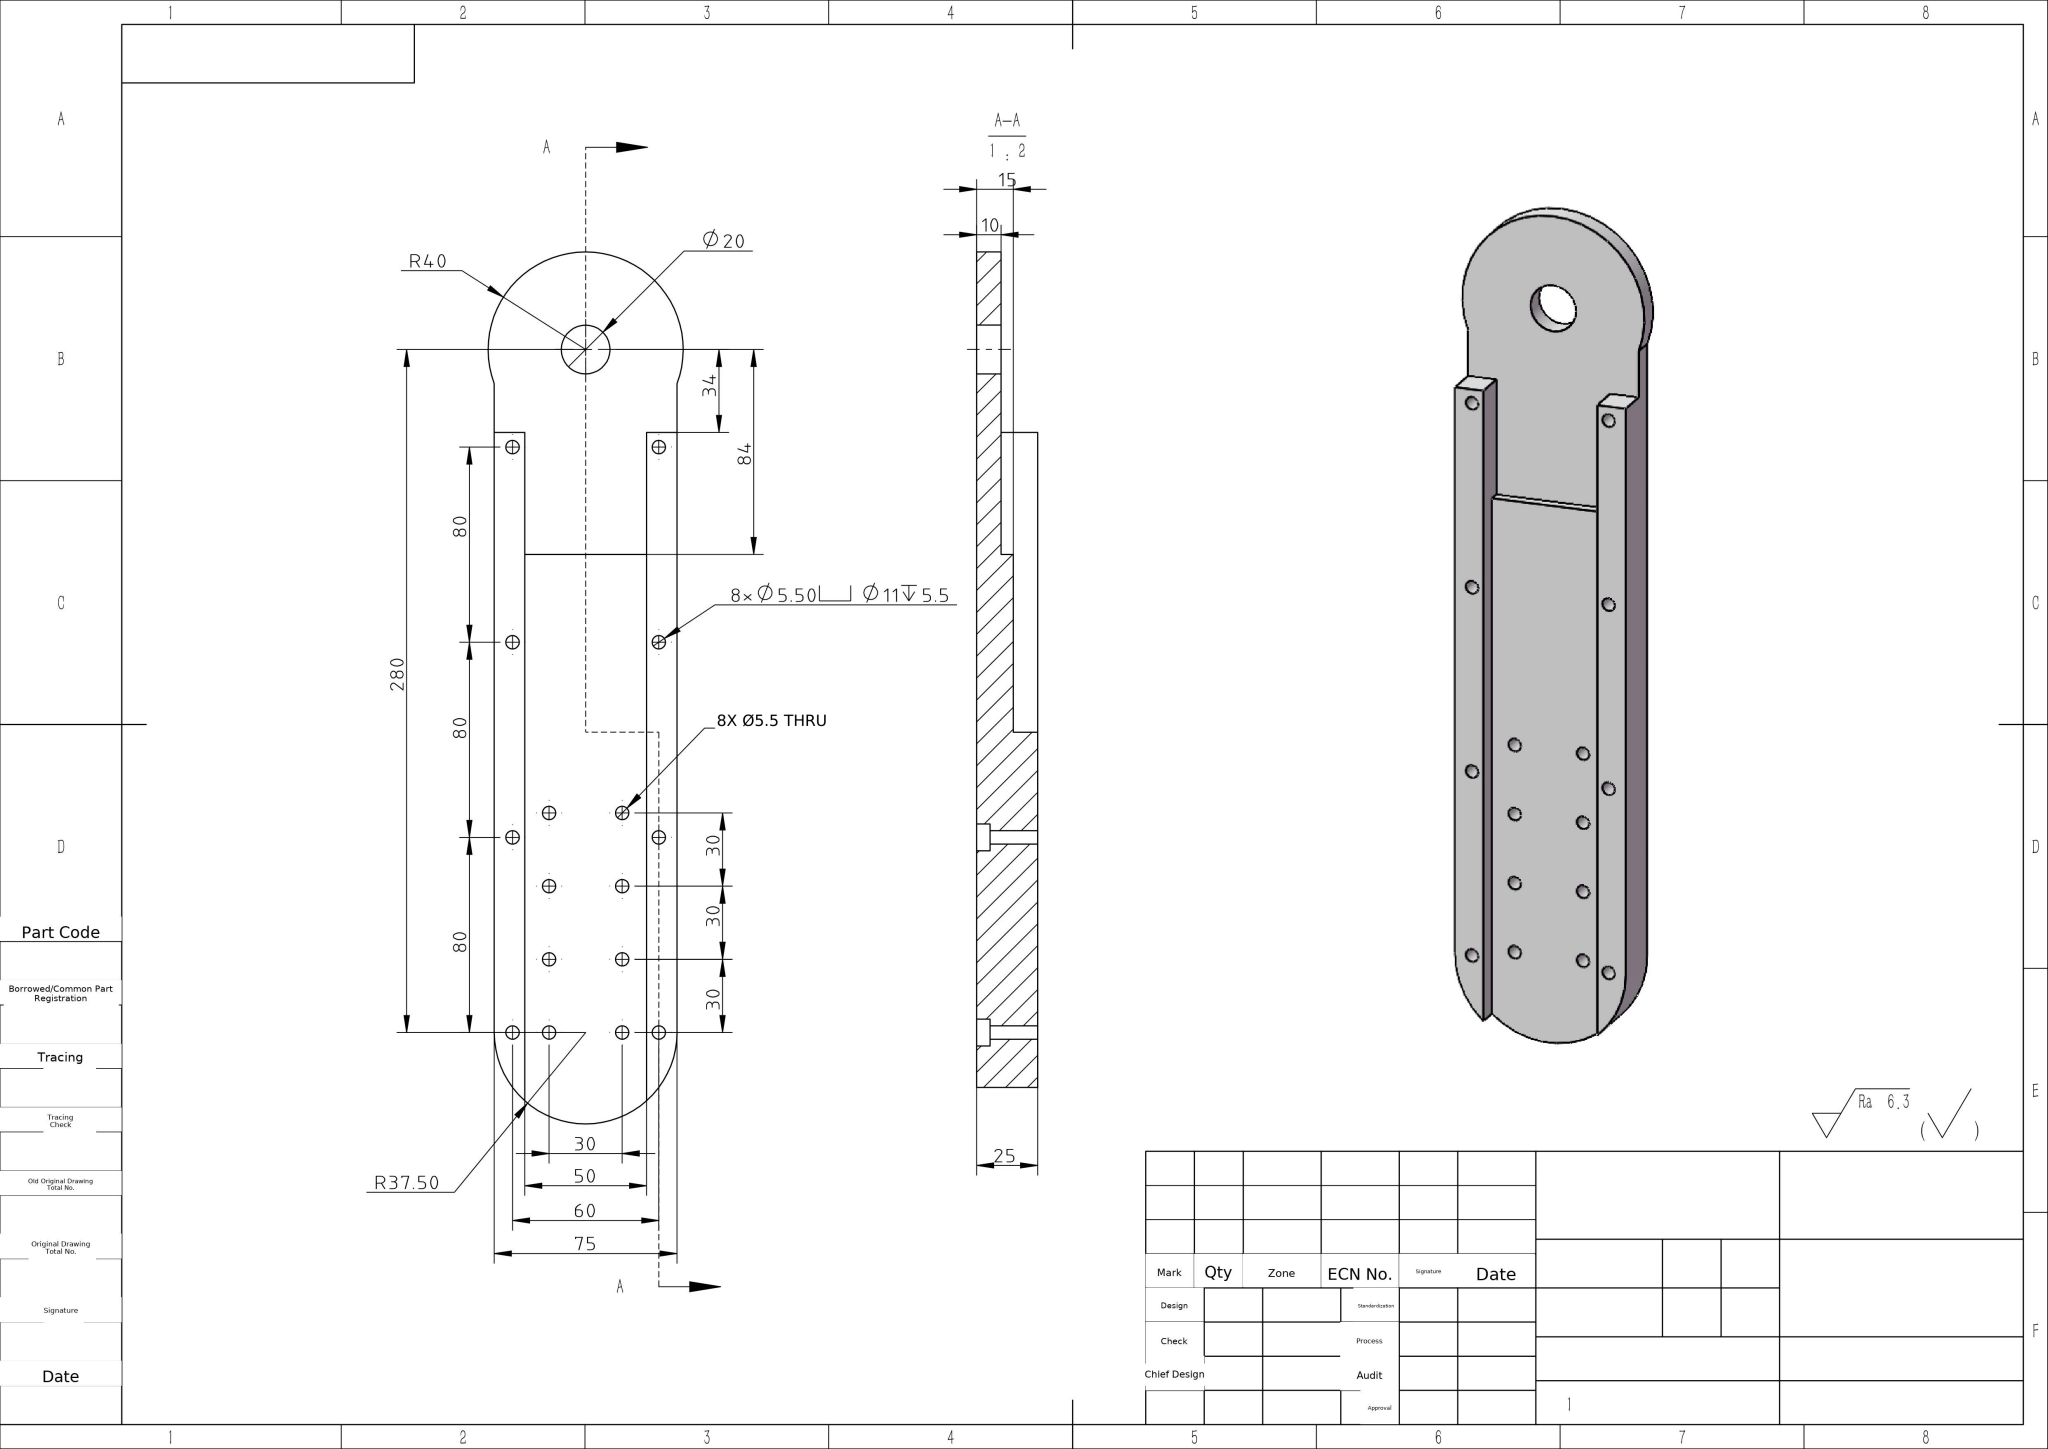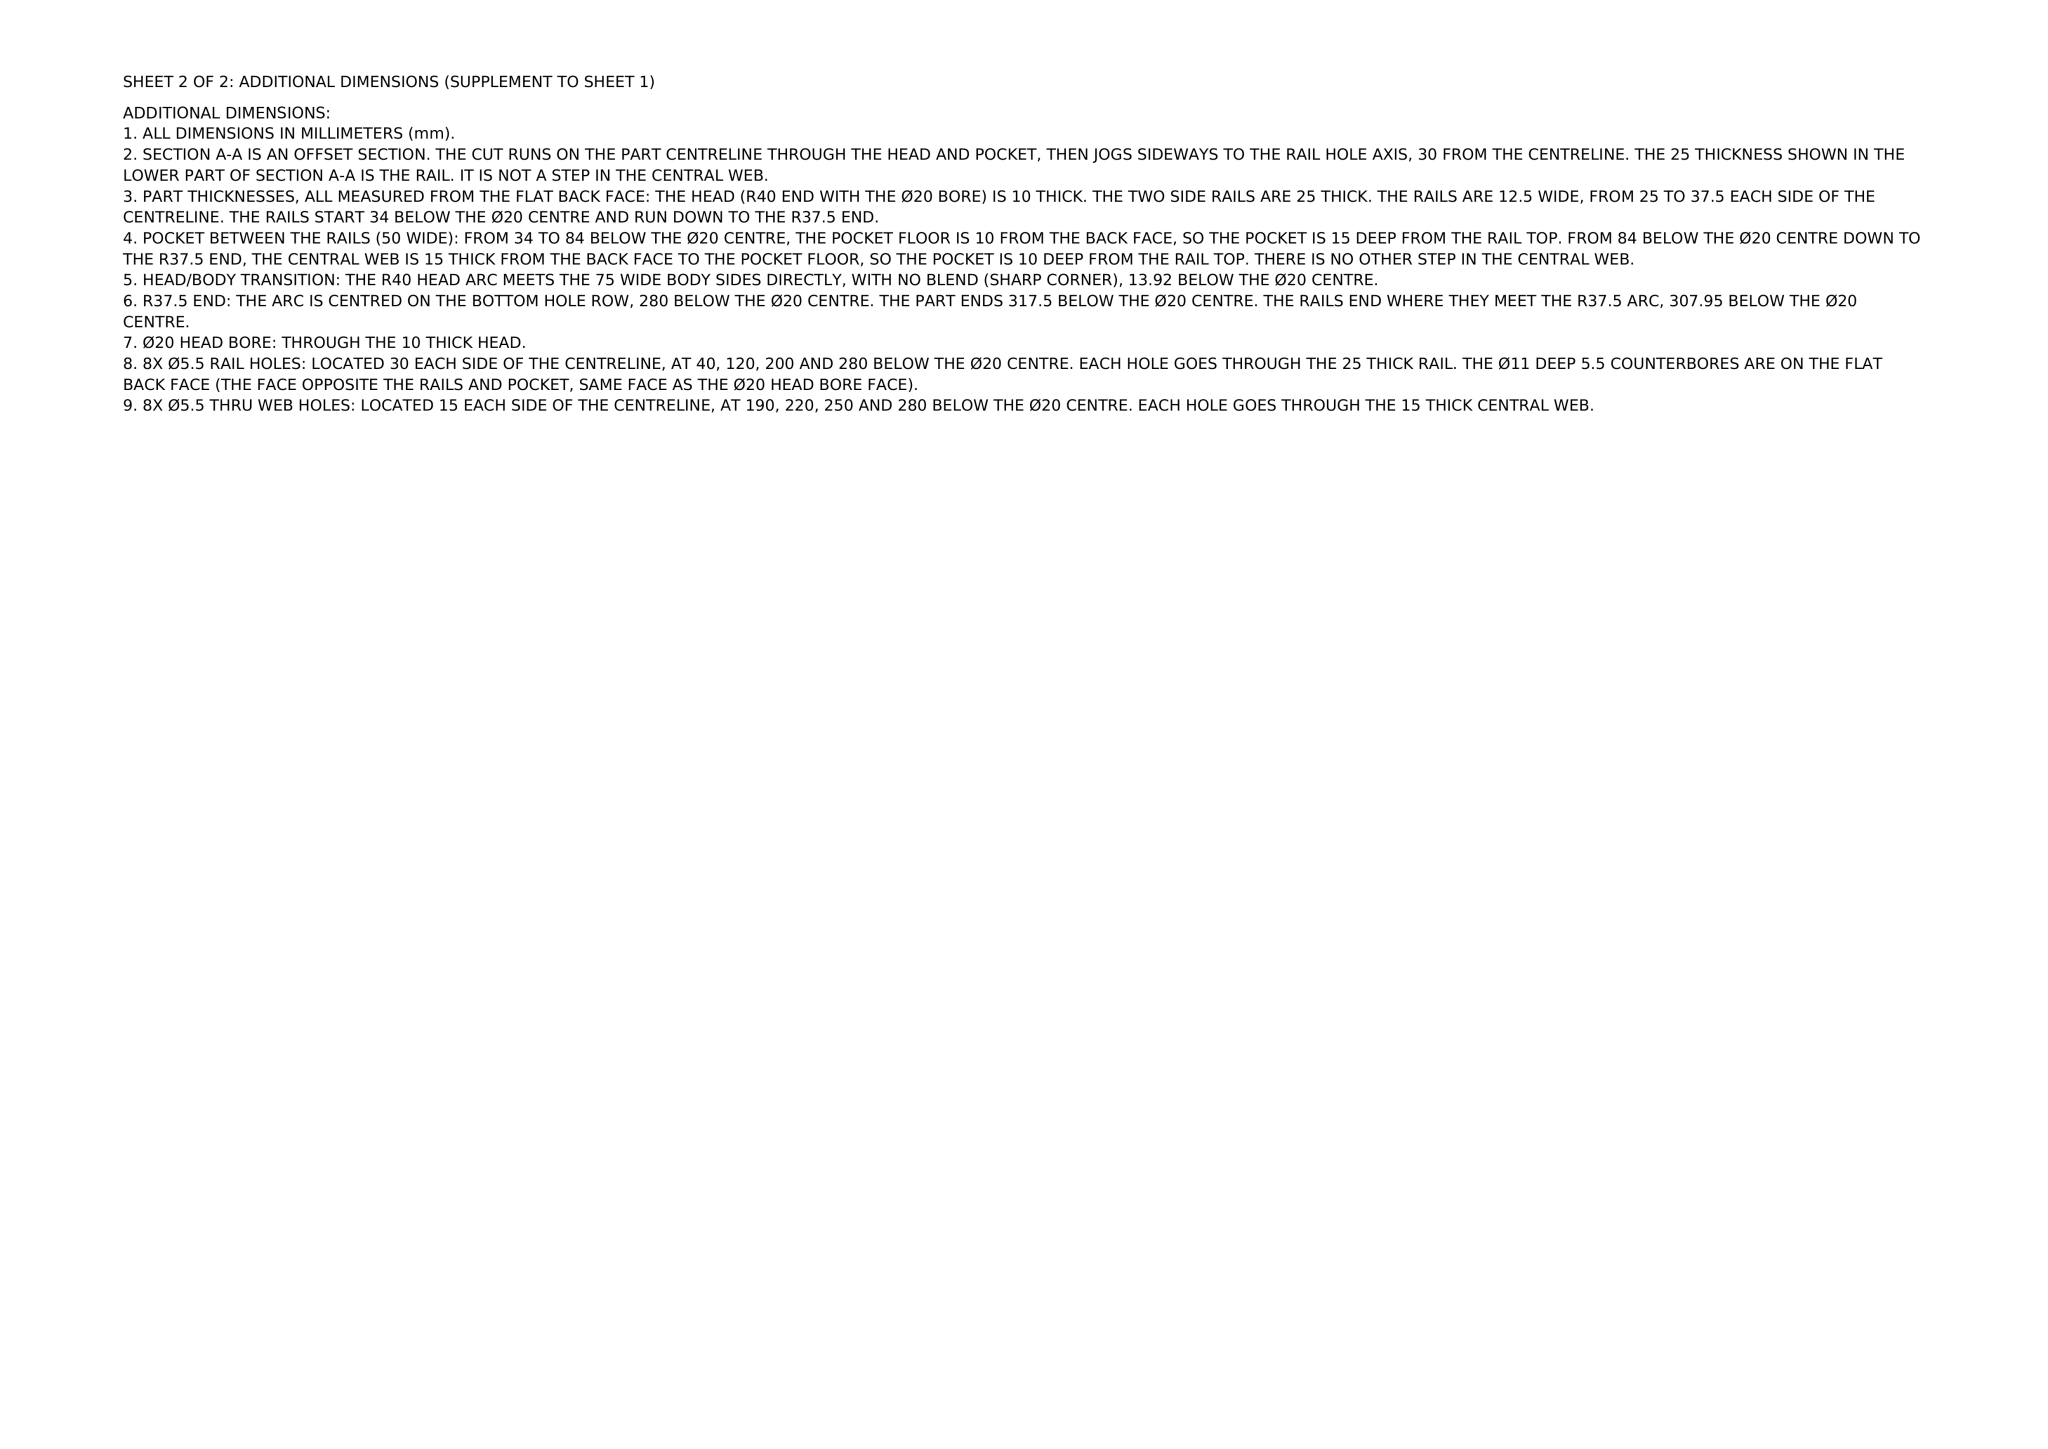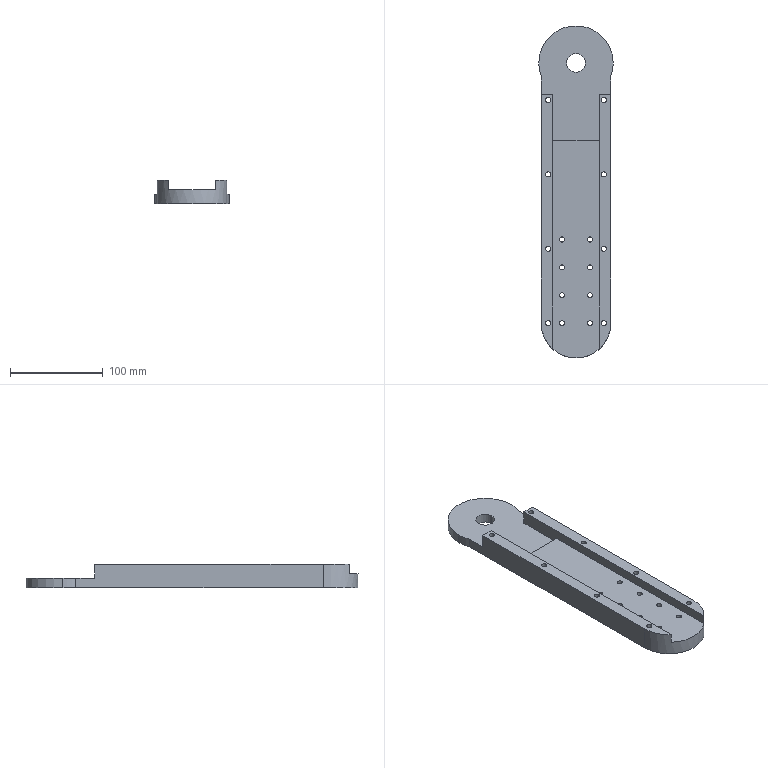Part | NX | mm | 1 solid | 74 faces | box 80 x 357.5 x 25 mm | volume 400943 mm3 | cylinder 54 | plane 20 | commonest cylinder face diameters 5.5 x32 11 x16 80 x3 20 x2 75 x1